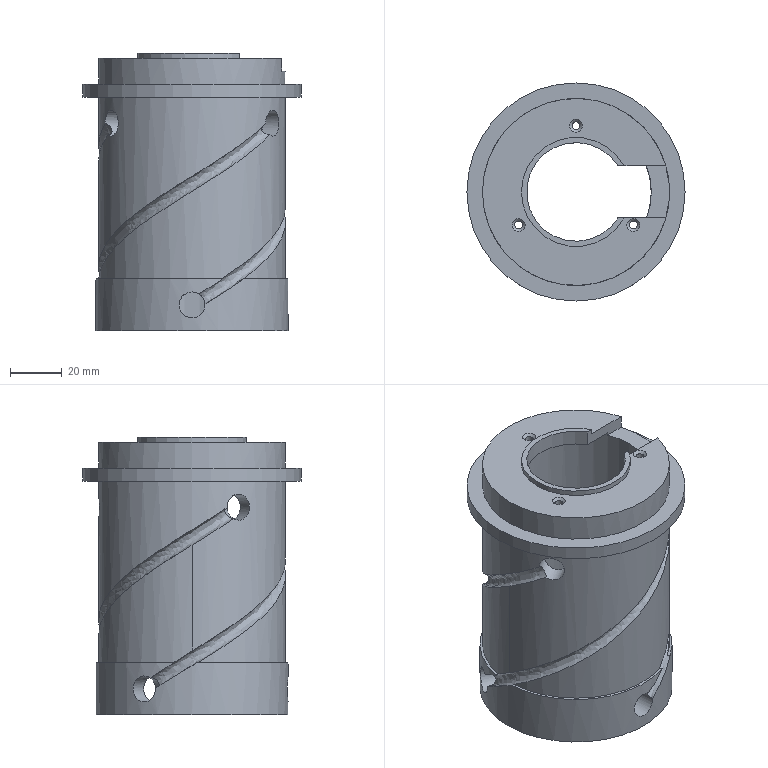CAM job | NX | mm | 3-axis | 1 set-up | 1 operations | part box 84 x 84 x 107
set-up 1
1. Cavity Milling | Mill Mill5 MILL_D10 | CAVITY_MILL | path 333036.879 mm | 412.877 min